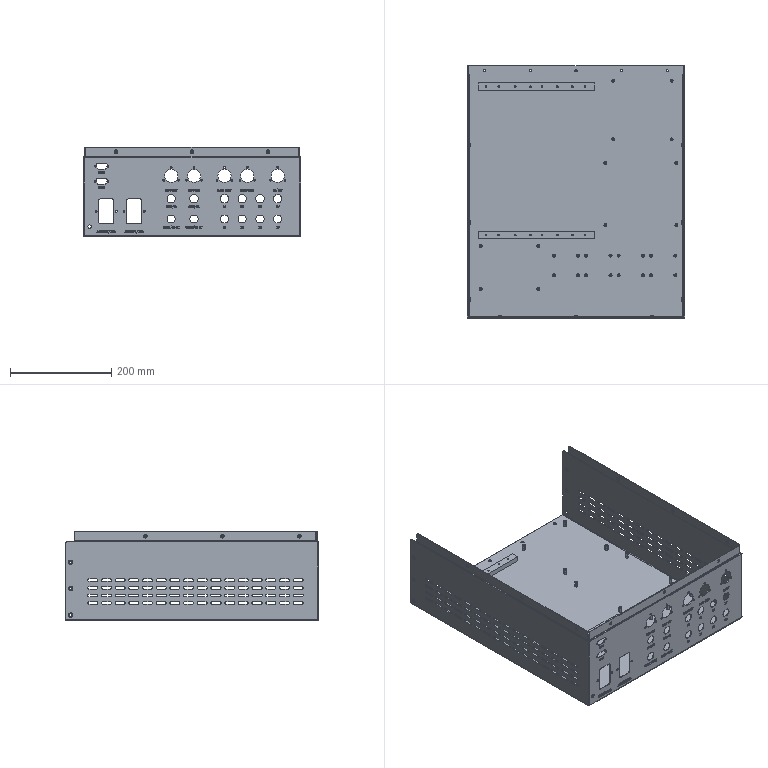CAM job | Mastercam | mm | 3 operations | part box 428 x 498.5 x 176.5
1. Contour (Ramp) | 8 - 8 平铣刀
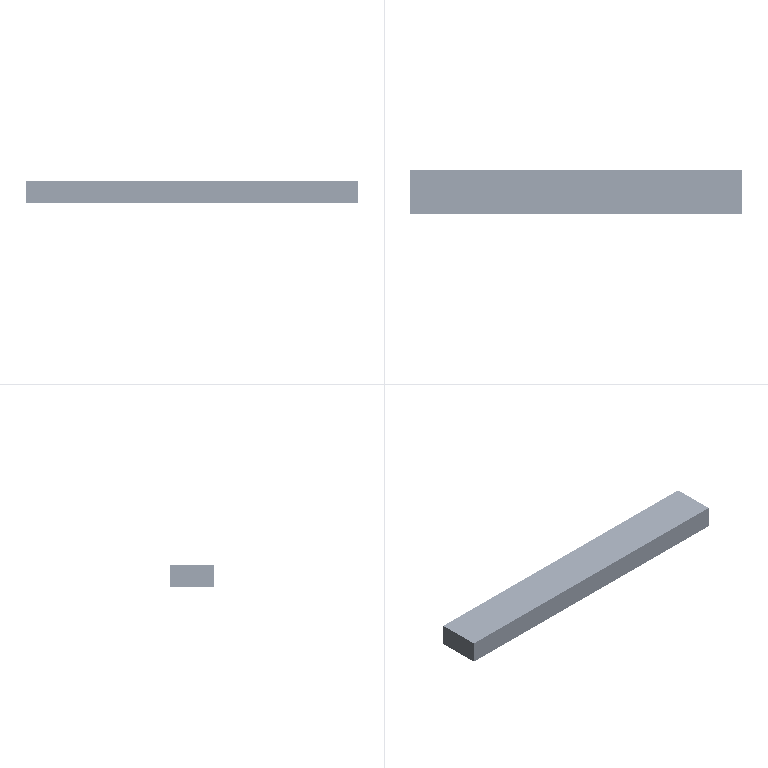2. Contour (2D) | 8 - 8 平铣刀
3. Drill/Counterbore | 7 - 4 倒角刀